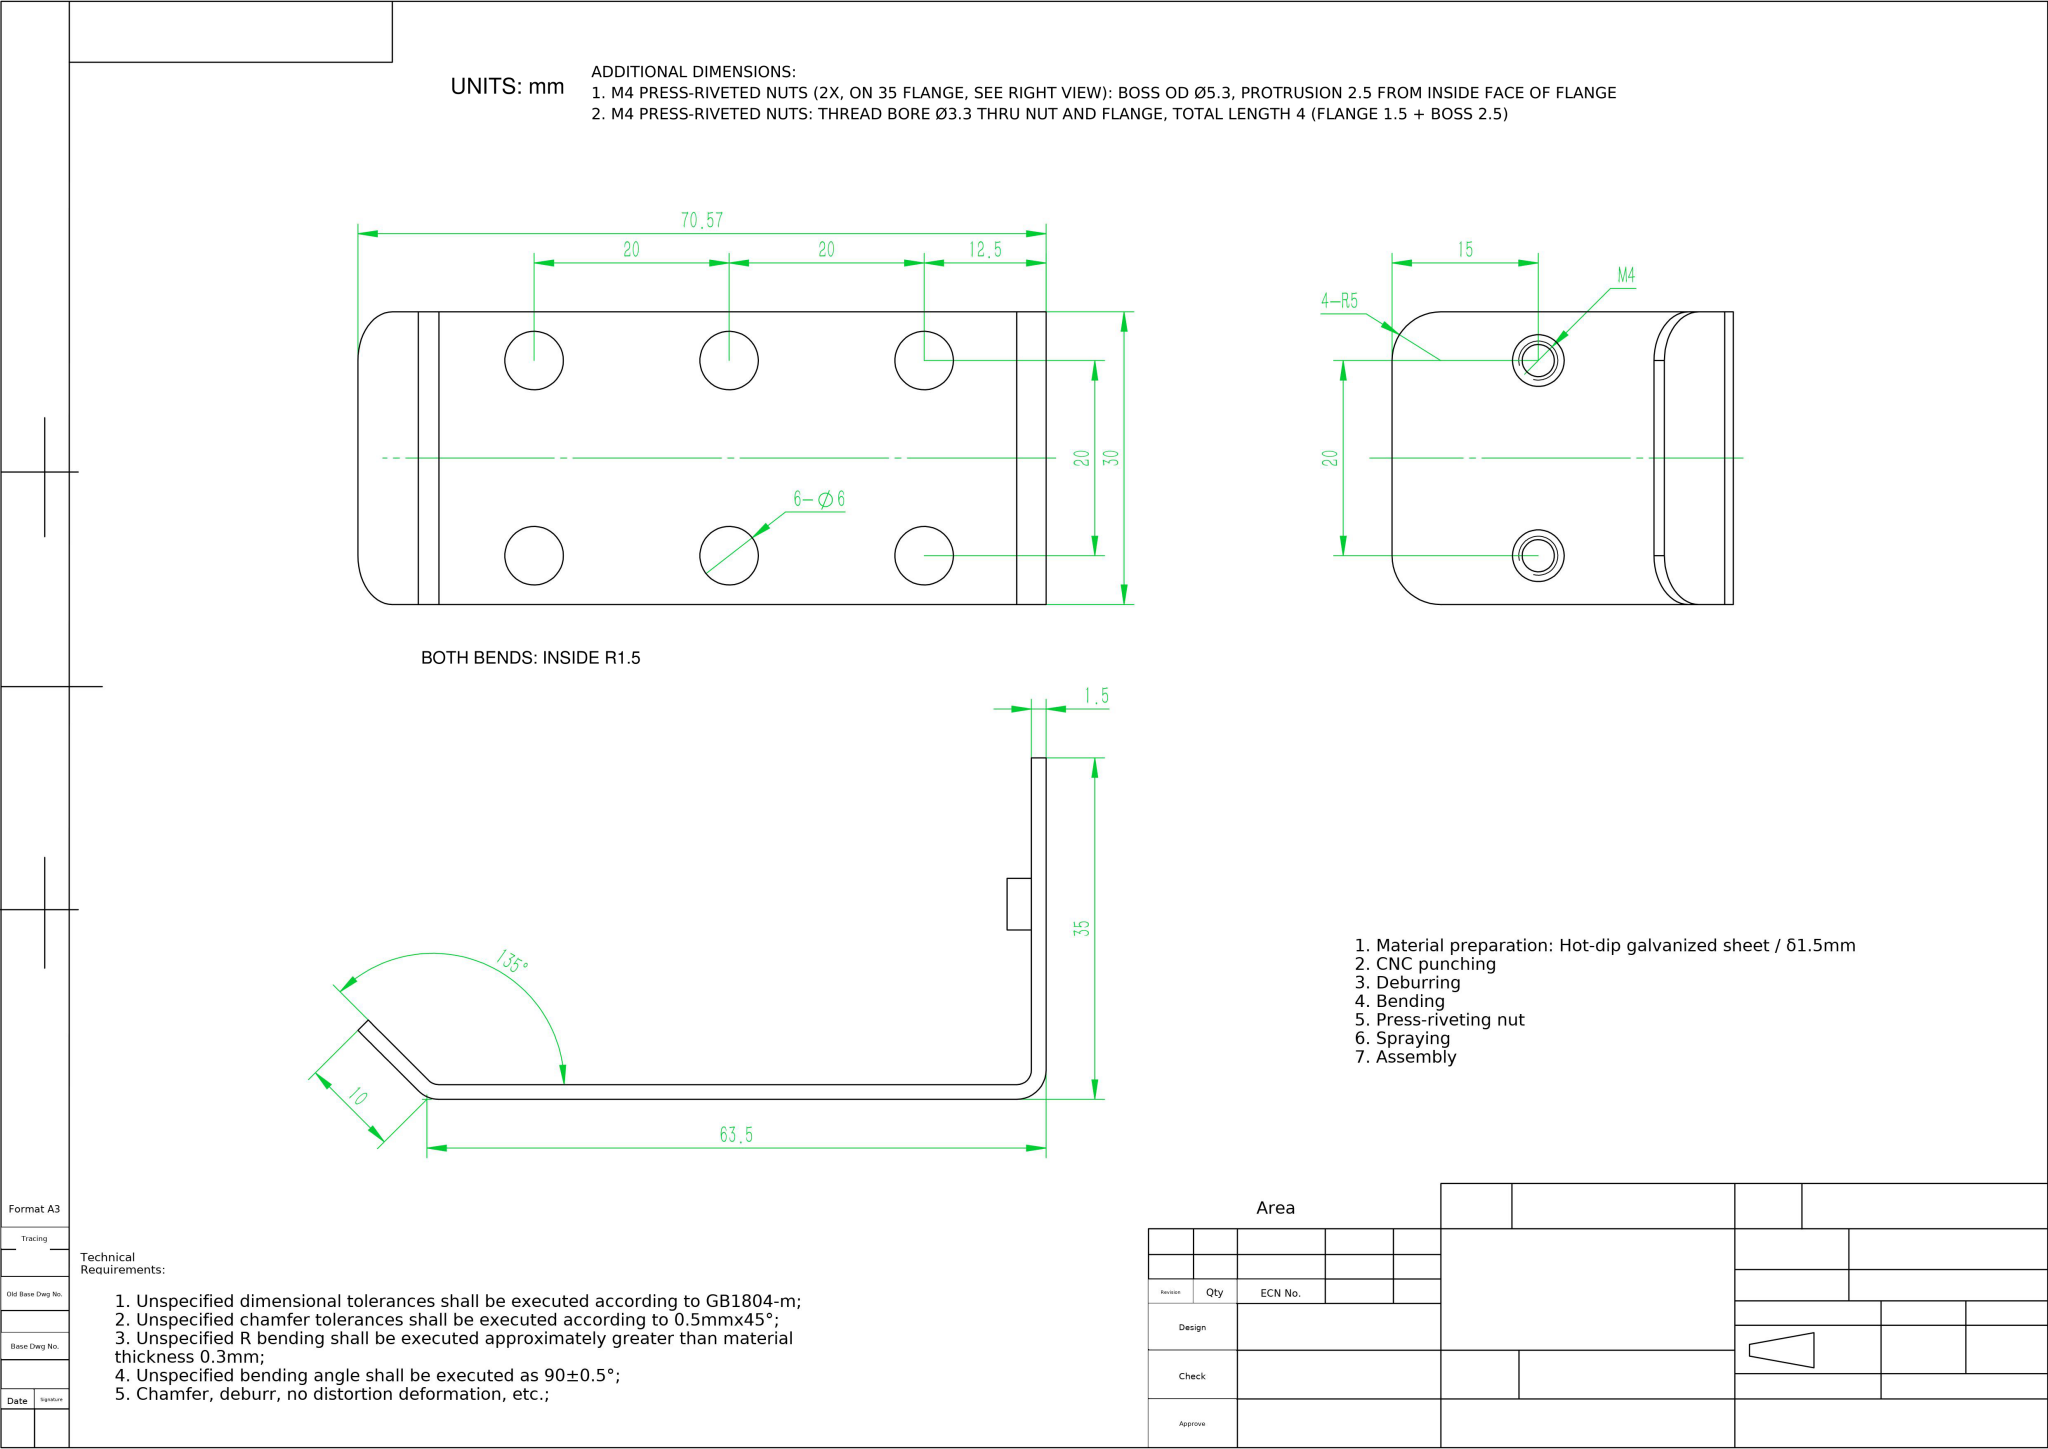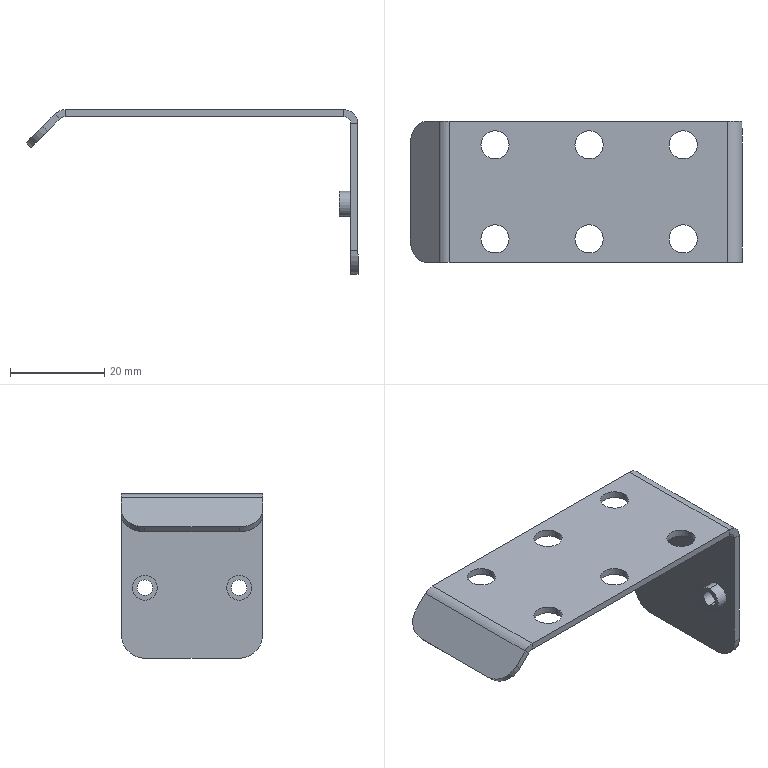Part | NX | mm | 1 solid | 48 faces | box 70.57 x 30 x 35 mm | volume 4494 mm3 | cylinder 28 | plane 20 | commonest cylinder face diameters 6 x14 3.3 x4 5.3 x4 10 x4 3 x2